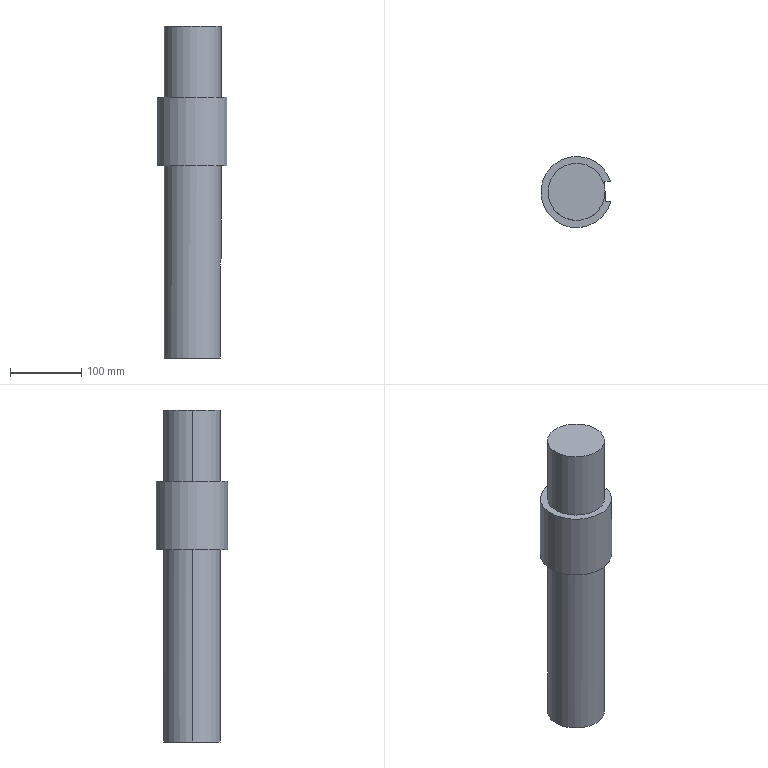Component | SolidWorks | 17WormGearShaft-1 | 1 solid | 16 faces | box 98.3 x 100 x 466 mm | volume 2562970 mm3 | plane 10 | cylinder 6 | commonest cylinder face diameters 80 x4 100 x1 22 x1
build123d program:
from build123d import *

# Parameters (mm, degrees)
SKETCH31_R          = 40
BOSS_EXTRUDE6_DEPTH = 466
BOSS_EXTRUDE9_START = -100
BOSS_EXTRUDE9_DEPTH = 96
CUT_EXTRUDE3_START  = 40
CUT_EXTRUDE3_DEPTH  = 9


with BuildPart() as part:
    # Sketch31 → Boss-Extrude6 (new body)
    with BuildSketch(Plane(origin=(0, 0, 0), x_dir=(0, 0, -1), z_dir=(1, 0, 0))):
        Circle(SKETCH31_R)
    extrude(amount=BOSS_EXTRUDE6_DEPTH)

    # Sketch32 → Boss-Extrude9 (add)
    with BuildSketch(Plane.ZY.offset(BOSS_EXTRUDE9_START)):
        with BuildLine():
            Line((48, 14), (40, 14))
            Line((40, 14), (40, -14))
            Line((40, -14), (48, -14))
            ThreePointArc((48, -14), (-50, 0), (48, 14))
        make_face()
    extrude(amount=-BOSS_EXTRUDE9_DEPTH)

    # Sketch33 → Cut-Extrude3 (cut)
    with BuildSketch(Plane.XY.offset(CUT_EXTRUDE3_START)):
        with BuildLine():
            Line((337, 11), (519.187, 11))
            ThreePointArc((519.187, 11), (530.187, 0), (519.187, -11))
            Line((519.187, -11), (337, -11))
            ThreePointArc((337, -11), (326, 0), (337, 11))
        make_face()
    extrude(amount=-CUT_EXTRUDE3_DEPTH, mode=Mode.SUBTRACT)


solid = part.part

# Placed as in the assembly
solid = solid.moved(Location((39.885, 141.809, 660), (-90, 88.714, 90)))
STEP:
#1=COLOUR_RGB('',0.7922,0.8196,0.9333);
#2=FILL_AREA_STYLE_COLOUR('',#1);
#3=FILL_AREA_STYLE('',(#2));
#4=SURFACE_STYLE_FILL_AREA(#3);
#5=SURFACE_SIDE_STYLE('',(#4));
#6=SURFACE_STYLE_USAGE(.BOTH.,#5);
#7=PRESENTATION_STYLE_ASSIGNMENT((#6));
#8=CARTESIAN_POINT('',(3.145,5.618,22.047));
#9=VERTEX_POINT('',#8);
#10=CARTESIAN_POINT('',(-0.004145,5.548,22.047));
#11=VERTEX_POINT('',#10);
#12=CARTESIAN_POINT('',(1.57,5.583,22.047));
#13=DIRECTION('',(0.,0.,1.));
#14=DIRECTION('',(0.9997,0.02244,0.));
#15=AXIS2_PLACEMENT_3D('',#12,#13,#14);
#16=CIRCLE('',#15,1.575);
#17=EDGE_CURVE('',#9,#11,#16,.T.);
#18=ORIENTED_EDGE('',*,*,#17,.T.);
#19=CARTESIAN_POINT('',(-0.004145,5.548,25.984));
#20=VERTEX_POINT('',#19);
#21=CARTESIAN_POINT('',(-0.004145,5.548,7.638));
#22=DIRECTION('',(0.,0.,1.));
#23=VECTOR('',#22,39.37);
#24=LINE('',#21,#23);
#25=EDGE_CURVE('',#11,#20,#24,.T.);
#26=ORIENTED_EDGE('',*,*,#25,.T.);
#27=CARTESIAN_POINT('',(3.145,5.618,25.984));
#28=VERTEX_POINT('',#27);
#29=CARTESIAN_POINT('',(1.57,5.583,25.984));
#30=DIRECTION('',(0.,0.,-1.));
#31=DIRECTION('',(-0.9997,-0.02244,0.));
#32=AXIS2_PLACEMENT_3D('',#29,#30,#31);
#33=CIRCLE('',#32,1.575);
#34=EDGE_CURVE('',#20,#28,#33,.T.);
#35=ORIENTED_EDGE('',*,*,#34,.T.);
#36=CARTESIAN_POINT('',(3.145,5.618,7.638));
#37=DIRECTION('',(0.,0.,1.));
#38=VECTOR('',#37,39.37);
#39=LINE('',#36,#38);
#40=EDGE_CURVE('',#9,#28,#39,.T.);
#41=ORIENTED_EDGE('',*,*,#40,.F.);
#42=EDGE_LOOP('',(#18,#26,#35,#41));
#43=FACE_OUTER_BOUND('',#42,.T.);
#44=CARTESIAN_POINT('',(1.57,5.583,7.638));
#45=DIRECTION('',(0.,0.,1.));
#46=DIRECTION('',(0.9997,0.02244,0.));
#47=AXIS2_PLACEMENT_3D('',#44,#45,#46);
#48=CYLINDRICAL_SURFACE('',#47,1.575);
#49=ADVANCED_FACE('',(#43),#48,.T.);
#50=CARTESIAN_POINT('',(-0.004145,5.548,7.638));
#51=VERTEX_POINT('',#50);
#52=CARTESIAN_POINT('',(3.074,6.05,7.638));
#53=VERTEX_POINT('',#52);
#54=CARTESIAN_POINT('',(1.57,5.583,7.638));
#55=DIRECTION('',(0.,0.,-1.));
#56=DIRECTION('',(-0.9997,-0.02244,0.));
#57=AXIS2_PLACEMENT_3D('',#54,#55,#56);
#58=CIRCLE('',#57,1.575);
#59=EDGE_CURVE('',#51,#53,#58,.T.);
#60=ORIENTED_EDGE('',*,*,#59,.F.);
#61=CARTESIAN_POINT('',(-0.004145,5.548,18.268));
#62=VERTEX_POINT('',#61);
#63=CARTESIAN_POINT('',(-0.004145,5.548,7.638));
#64=DIRECTION('',(0.,0.,1.));
#65=VECTOR('',#64,39.37);
#66=LINE('',#63,#65);
#67=EDGE_CURVE('',#51,#62,#66,.T.);
#68=ORIENTED_EDGE('',*,*,#67,.T.);
#69=CARTESIAN_POINT('',(3.145,5.618,18.268));
#70=VERTEX_POINT('',#69);
#71=CARTESIAN_POINT('',(1.57,5.583,18.268));
#72=DIRECTION('',(0.,0.,1.));
#73=DIRECTION('',(0.9997,0.02244,0.));
#74=AXIS2_PLACEMENT_3D('',#71,#72,#73);
#75=CIRCLE('',#74,1.575);
#76=EDGE_CURVE('',#70,#62,#75,.T.);
#77=ORIENTED_EDGE('',*,*,#76,.F.);
#78=CARTESIAN_POINT('',(3.145,5.618,13.15));
#79=VERTEX_POINT('',#78);
#80=CARTESIAN_POINT('',(3.145,5.618,7.638));
#81=DIRECTION('',(0.,0.,1.));
#82=VECTOR('',#81,39.37);
#83=LINE('',#80,#82);
#84=EDGE_CURVE('',#79,#70,#83,.T.);
#85=ORIENTED_EDGE('',*,*,#84,.F.);
#86=CARTESIAN_POINT('',(3.074,6.05,12.717));
#87=VERTEX_POINT('',#86);
#88=CARTESIAN_POINT('',(3.145,5.618,13.15));
#89=CARTESIAN_POINT('',(3.144,5.647,13.15));
#90=CARTESIAN_POINT('',(3.143,5.676,13.147));
#91=CARTESIAN_POINT('',(3.138,5.731,13.136));
#92=CARTESIAN_POINT('',(3.136,5.758,13.127));
#93=CARTESIAN_POINT('',(3.13,5.797,13.111));
#94=CARTESIAN_POINT('',(3.129,5.81,13.105));
#95=CARTESIAN_POINT('',(3.125,5.835,13.092));
#96=CARTESIAN_POINT('',(3.123,5.847,13.084));
#97=CARTESIAN_POINT('',(3.119,5.87,13.069));
#98=CARTESIAN_POINT('',(3.117,5.882,13.06));
#99=CARTESIAN_POINT('',(3.112,5.903,13.042));
#100=CARTESIAN_POINT('',(3.11,5.914,13.033));
#101=CARTESIAN_POINT('',(3.103,5.944,13.003));
#102=CARTESIAN_POINT('',(3.099,5.962,12.981));
#103=CARTESIAN_POINT('',(3.093,5.985,12.946));
#104=CARTESIAN_POINT('',(3.091,5.992,12.934));
#105=CARTESIAN_POINT('',(3.087,6.006,12.909));
#106=CARTESIAN_POINT('',(3.086,6.012,12.896));
#107=CARTESIAN_POINT('',(3.081,6.028,12.857));
#108=CARTESIAN_POINT('',(3.079,6.036,12.83));
#109=CARTESIAN_POINT('',(3.076,6.044,12.788));
#110=CARTESIAN_POINT('',(3.075,6.046,12.774));
#111=CARTESIAN_POINT('',(3.074,6.049,12.745));
#112=CARTESIAN_POINT('',(3.074,6.05,12.731));
#113=CARTESIAN_POINT('',(3.074,6.05,12.717));
#114=B_SPLINE_CURVE_WITH_KNOTS('',3,(#88,#89,#90,#91,#92,#93,#94,#95,#96,#97,#98,#99,#100,#101,#102,#103,#104,#105,#106,#107,#108,#109,#110,#111,#112,#113),.UNSPECIFIED.,.F.,.F.,(4,2,2,2,2,2,2,2,2,2,2,2,4),(0.01728,0.01944,0.0216,0.02268,0.02376,0.02484,0.02592,0.02807,0.02915,0.03023,0.03239,0.03347,0.03455),.UNSPECIFIED.);
#115=EDGE_CURVE('',#79,#87,#114,.T.);
#116=ORIENTED_EDGE('',*,*,#115,.T.);
#117=CARTESIAN_POINT('',(3.074,6.05,7.638));
#118=DIRECTION('',(0.,0.,-1.));
#119=VECTOR('',#118,39.37);
#120=LINE('',#117,#119);
#121=EDGE_CURVE('',#87,#53,#120,.T.);
#122=ORIENTED_EDGE('',*,*,#121,.T.);
#123=EDGE_LOOP('',(#60,#68,#77,#85,#116,#122));
#124=FACE_OUTER_BOUND('',#123,.T.);
#125=CARTESIAN_POINT('',(1.57,5.583,7.638));
#126=DIRECTION('',(0.,0.,1.));
#127=DIRECTION('',(0.9997,0.02244,0.));
#128=AXIS2_PLACEMENT_3D('',#125,#126,#127);
#129=CYLINDRICAL_SURFACE('',#128,1.575);
#130=ADVANCED_FACE('',(#124),#129,.T.);
#131=ORIENTED_EDGE('',*,*,#67,.F.);
#132=CARTESIAN_POINT('',(3.094,5.184,7.638));
#133=VERTEX_POINT('',#132);
#134=CARTESIAN_POINT('',(1.57,5.583,7.638));
#135=DIRECTION('',(0.,0.,-1.));
#136=DIRECTION('',(-0.9997,-0.02244,0.));
#137=AXIS2_PLACEMENT_3D('',#134,#135,#136);
#138=CIRCLE('',#137,1.575);
#139=EDGE_CURVE('',#133,#51,#138,.T.);
#140=ORIENTED_EDGE('',*,*,#139,.F.);
#141=CARTESIAN_POINT('',(3.094,5.184,12.717));
#142=VERTEX_POINT('',#141);
#143=CARTESIAN_POINT('',(3.094,5.184,7.638));
#144=DIRECTION('',(0.,0.,1.));
#145=VECTOR('',#144,39.37);
#146=LINE('',#143,#145);
#147=EDGE_CURVE('',#133,#142,#146,.T.);
#148=ORIENTED_EDGE('',*,*,#147,.T.);
#149=CARTESIAN_POINT('',(3.094,5.184,12.717));
#150=CARTESIAN_POINT('',(3.094,5.184,12.745));
#151=CARTESIAN_POINT('',(3.094,5.187,12.774));
#152=CARTESIAN_POINT('',(3.097,5.195,12.815));
#153=CARTESIAN_POINT('',(3.097,5.199,12.829));
#154=CARTESIAN_POINT('',(3.1,5.207,12.856));
#155=CARTESIAN_POINT('',(3.101,5.212,12.87));
#156=CARTESIAN_POINT('',(3.105,5.228,12.909));
#157=CARTESIAN_POINT('',(3.108,5.242,12.934));
#158=CARTESIAN_POINT('',(3.113,5.266,12.969));
#159=CARTESIAN_POINT('',(3.114,5.274,12.981));
#160=CARTESIAN_POINT('',(3.118,5.292,13.003));
#161=CARTESIAN_POINT('',(3.12,5.302,13.013));
#162=CARTESIAN_POINT('',(3.125,5.332,13.043));
#163=CARTESIAN_POINT('',(3.128,5.353,13.061));
#164=CARTESIAN_POINT('',(3.133,5.389,13.084));
#165=CARTESIAN_POINT('',(3.135,5.401,13.092));
#166=CARTESIAN_POINT('',(3.137,5.426,13.105));
#167=CARTESIAN_POINT('',(3.139,5.439,13.111));
#168=CARTESIAN_POINT('',(3.141,5.465,13.122));
#169=CARTESIAN_POINT('',(3.142,5.478,13.127));
#170=CARTESIAN_POINT('',(3.143,5.506,13.135));
#171=CARTESIAN_POINT('',(3.144,5.52,13.138));
#172=CARTESIAN_POINT('',(3.145,5.562,13.147));
#173=CARTESIAN_POINT('',(3.145,5.59,13.15));
#174=CARTESIAN_POINT('',(3.145,5.618,13.15));
#175=B_SPLINE_CURVE_WITH_KNOTS('',3,(#149,#150,#151,#152,#153,#154,#155,#156,#157,#158,#159,#160,#161,#162,#163,#164,#165,#166,#167,#168,#169,#170,#171,#172,#173,#174),.UNSPECIFIED.,.F.,.F.,(4,2,2,2,2,2,2,2,2,2,2,2,4),(0.,0.00216,0.003241,0.004321,0.006481,0.007562,0.008642,0.0108,0.01188,0.01296,0.01404,0.01512,0.01728),.UNSPECIFIED.);
#176=EDGE_CURVE('',#142,#79,#175,.T.);
#177=ORIENTED_EDGE('',*,*,#176,.T.);
#178=ORIENTED_EDGE('',*,*,#84,.T.);
#179=CARTESIAN_POINT('',(1.57,5.583,18.268));
#180=DIRECTION('',(0.,0.,1.));
#181=DIRECTION('',(0.9997,0.02244,0.));
#182=AXIS2_PLACEMENT_3D('',#179,#180,#181);
#183=CIRCLE('',#182,1.575);
#184=EDGE_CURVE('',#62,#70,#183,.T.);
#185=ORIENTED_EDGE('',*,*,#184,.F.);
#186=EDGE_LOOP('',(#131,#140,#148,#177,#178,#185));
#187=FACE_OUTER_BOUND('',#186,.T.);
#188=CARTESIAN_POINT('',(1.57,5.583,7.638));
#189=DIRECTION('',(0.,0.,1.));
#190=DIRECTION('',(0.9997,0.02244,0.));
#191=AXIS2_PLACEMENT_3D('',#188,#189,#190);
#192=CYLINDRICAL_SURFACE('',#191,1.575);
#193=ADVANCED_FACE('',(#187),#192,.T.);
#194=CARTESIAN_POINT('',(2.781,6.043,7.638));
#195=VERTEX_POINT('',#194);
#196=CARTESIAN_POINT('',(1.561,6.016,7.638));
#197=DIRECTION('',(0.9997,0.02244,0.));
#198=VECTOR('',#197,39.37);
#199=LINE('',#196,#198);
#200=EDGE_CURVE('',#195,#53,#199,.T.);
#201=ORIENTED_EDGE('',*,*,#200,.F.);
#202=CARTESIAN_POINT('',(2.8,5.177,7.638));
#203=VERTEX_POINT('',#202);
#204=CARTESIAN_POINT('',(2.79,5.61,7.638));
#205=DIRECTION('',(0.02244,-0.9997,0.));
#206=VECTOR('',#205,39.37);
#207=LINE('',#204,#206);
#208=EDGE_CURVE('',#195,#203,#207,.T.);
#209=ORIENTED_EDGE('',*,*,#208,.T.);
#210=CARTESIAN_POINT('',(1.58,5.15,7.638));
#211=DIRECTION('',(-0.9997,-0.02244,0.));
#212=VECTOR('',#211,39.37);
#213=LINE('',#210,#212);
#214=EDGE_CURVE('',#133,#203,#213,.T.);
#215=ORIENTED_EDGE('',*,*,#214,.F.);
#216=ORIENTED_EDGE('',*,*,#139,.T.);
#217=ORIENTED_EDGE('',*,*,#59,.T.);
#218=EDGE_LOOP('',(#201,#209,#215,#216,#217));
#219=FACE_OUTER_BOUND('',#218,.T.);
#220=CARTESIAN_POINT('',(1.57,5.583,7.638));
#221=DIRECTION('',(0.,0.,-1.));
#222=DIRECTION('',(-0.9997,-0.02244,0.));
#223=AXIS2_PLACEMENT_3D('',#220,#221,#222);
#224=PLANE('',#223);
#225=ADVANCED_FACE('',(#219),#224,.T.);
#226=CARTESIAN_POINT('',(3.157,5.067,18.268));
#227=VERTEX_POINT('',#226);
#228=CARTESIAN_POINT('',(3.132,6.169,18.268));
#229=DIRECTION('',(0.02244,-0.9997,0.));
#230=VECTOR('',#229,39.37);
#231=LINE('',#228,#230);
#232=EDGE_CURVE('',#70,#227,#231,.T.);
#233=ORIENTED_EDGE('',*,*,#232,.F.);
#234=CARTESIAN_POINT('',(3.132,6.169,18.268));
#235=VERTEX_POINT('',#234);
#236=CARTESIAN_POINT('',(3.132,6.169,18.268));
#237=DIRECTION('',(0.02244,-0.9997,0.));
#238=VECTOR('',#237,39.37);
#239=LINE('',#236,#238);
#240=EDGE_CURVE('',#235,#70,#239,.T.);
#241=ORIENTED_EDGE('',*,*,#240,.F.);
#242=CARTESIAN_POINT('',(3.132,6.169,22.047));
#243=VERTEX_POINT('',#242);
#244=CARTESIAN_POINT('',(3.132,6.169,18.268));
#245=DIRECTION('',(0.,0.,1.));
#246=VECTOR('',#245,39.37);
#247=LINE('',#244,#246);
#248=EDGE_CURVE('',#235,#243,#247,.T.);
#249=ORIENTED_EDGE('',*,*,#248,.T.);
#250=CARTESIAN_POINT('',(3.132,6.169,22.047));
#251=DIRECTION('',(0.02244,-0.9997,0.));
#252=VECTOR('',#251,39.37);
#253=LINE('',#250,#252);
#254=EDGE_CURVE('',#243,#9,#253,.T.);
#255=ORIENTED_EDGE('',*,*,#254,.T.);
#256=CARTESIAN_POINT('',(3.157,5.067,22.047));
#257=VERTEX_POINT('',#256);
#258=CARTESIAN_POINT('',(3.132,6.169,22.047));
#259=DIRECTION('',(0.02244,-0.9997,0.));
#260=VECTOR('',#259,39.37);
#261=LINE('',#258,#260);
#262=EDGE_CURVE('',#9,#257,#261,.T.);
#263=ORIENTED_EDGE('',*,*,#262,.T.);
#264=CARTESIAN_POINT('',(3.157,5.067,18.268));
#265=DIRECTION('',(0.,0.,1.));
#266=VECTOR('',#265,39.37);
#267=LINE('',#264,#266);
#268=EDGE_CURVE('',#227,#257,#267,.T.);
#269=ORIENTED_EDGE('',*,*,#268,.F.);
#270=EDGE_LOOP('',(#233,#241,#249,#255,#263,#269));
#271=FACE_OUTER_BOUND('',#270,.T.);
#272=CARTESIAN_POINT('',(3.132,6.169,18.268));
#273=DIRECTION('',(-0.9997,-0.02244,0.));
#274=DIRECTION('',(0.,0.,1.));
#275=AXIS2_PLACEMENT_3D('',#272,#273,#274);
#276=PLANE('',#275);
#277=ADVANCED_FACE('',(#271),#276,.F.);
#278=CARTESIAN_POINT('',(3.447,6.176,22.047));
#279=VERTEX_POINT('',#278);
#280=CARTESIAN_POINT('',(3.447,6.176,22.047));
#281=DIRECTION('',(-0.9997,-0.02244,0.));
#282=VECTOR('',#281,39.37);
#283=LINE('',#280,#282);
#284=EDGE_CURVE('',#279,#243,#283,.T.);
#285=ORIENTED_EDGE('',*,*,#284,.T.);
#286=ORIENTED_EDGE('',*,*,#248,.F.);
#287=CARTESIAN_POINT('',(3.447,6.176,18.268));
#288=VERTEX_POINT('',#287);
#289=CARTESIAN_POINT('',(3.447,6.176,18.268));
#290=DIRECTION('',(-0.9997,-0.02244,0.));
#291=VECTOR('',#290,39.37);
#292=LINE('',#289,#291);
#293=EDGE_CURVE('',#288,#235,#292,.T.);
#294=ORIENTED_EDGE('',*,*,#293,.F.);
#295=CARTESIAN_POINT('',(3.447,6.176,18.268));
#296=DIRECTION('',(0.,0.,1.));
#297=VECTOR('',#296,39.37);
#298=LINE('',#295,#297);
#299=EDGE_CURVE('',#288,#279,#298,.T.);
#300=ORIENTED_EDGE('',*,*,#299,.T.);
#301=EDGE_LOOP('',(#285,#286,#294,#300));
#302=FACE_OUTER_BOUND('',#301,.T.);
#303=CARTESIAN_POINT('',(3.447,6.176,18.268));
#304=DIRECTION('',(-0.02244,0.9997,0.));
#305=DIRECTION('',(0.9997,0.02244,0.));
#306=AXIS2_PLACEMENT_3D('',#303,#304,#305);
#307=PLANE('',#306);
#308=ADVANCED_FACE('',(#302),#307,.F.);
#309=CARTESIAN_POINT('',(3.472,5.074,22.047));
#310=VERTEX_POINT('',#309);
#311=CARTESIAN_POINT('',(3.472,5.074,22.047));
#312=DIRECTION('',(-0.9997,-0.02244,0.));
#313=VECTOR('',#312,39.37);
#314=LINE('',#311,#313);
#315=EDGE_CURVE('',#310,#257,#314,.T.);
#316=ORIENTED_EDGE('',*,*,#315,.F.);
#317=CARTESIAN_POINT('',(3.472,5.074,18.268));
#318=VERTEX_POINT('',#317);
#319=CARTESIAN_POINT('',(3.472,5.074,18.268));
#320=DIRECTION('',(0.,0.,1.));
#321=VECTOR('',#320,39.37);
#322=LINE('',#319,#321);
#323=EDGE_CURVE('',#318,#310,#322,.T.);
#324=ORIENTED_EDGE('',*,*,#323,.F.);
#325=CARTESIAN_POINT('',(3.472,5.074,18.268));
#326=DIRECTION('',(-0.9997,-0.02244,0.));
#327=VECTOR('',#326,39.37);
#328=LINE('',#325,#327);
#329=EDGE_CURVE('',#318,#227,#328,.T.);
#330=ORIENTED_EDGE('',*,*,#329,.T.);
#331=ORIENTED_EDGE('',*,*,#268,.T.);
#332=EDGE_LOOP('',(#316,#324,#330,#331));
#333=FACE_OUTER_BOUND('',#332,.T.);
#334=CARTESIAN_POINT('',(3.472,5.074,18.268));
#335=DIRECTION('',(-0.02244,0.9997,0.));
#336=DIRECTION('',(0.9997,0.02244,0.));
#337=AXIS2_PLACEMENT_3D('',#334,#335,#336);
#338=PLANE('',#337);
#339=ADVANCED_FACE('',(#333),#338,.T.);
#340=CARTESIAN_POINT('',(1.57,5.583,22.047));
#341=DIRECTION('',(0.,0.,1.));
#342=DIRECTION('',(0.9997,0.02244,0.));
#343=AXIS2_PLACEMENT_3D('',#340,#341,#342);
#344=CIRCLE('',#343,1.969);
#345=EDGE_CURVE('',#279,#310,#344,.T.);
#346=ORIENTED_EDGE('',*,*,#345,.F.);
#347=ORIENTED_EDGE('',*,*,#299,.F.);
#348=CARTESIAN_POINT('',(1.57,5.583,18.268));
#349=DIRECTION('',(0.,0.,1.));
#350=DIRECTION('',(0.9997,0.02244,0.));
#351=AXIS2_PLACEMENT_3D('',#348,#349,#350);
#352=CIRCLE('',#351,1.969);
#353=EDGE_CURVE('',#288,#318,#352,.T.);
#354=ORIENTED_EDGE('',*,*,#353,.T.);
#355=ORIENTED_EDGE('',*,*,#323,.T.);
#356=EDGE_LOOP('',(#346,#347,#354,#355));
#357=FACE_OUTER_BOUND('',#356,.T.);
#358=CARTESIAN_POINT('',(1.57,5.583,18.268));
#359=DIRECTION('',(0.,0.,1.));
#360=DIRECTION('',(0.9997,0.02244,0.));
#361=AXIS2_PLACEMENT_3D('',#358,#359,#360);
#362=CYLINDRICAL_SURFACE('',#361,1.969);
#363=ADVANCED_FACE('',(#357),#362,.T.);
#364=ORIENTED_EDGE('',*,*,#240,.T.);
#365=ORIENTED_EDGE('',*,*,#76,.T.);
#366=ORIENTED_EDGE('',*,*,#184,.T.);
#367=ORIENTED_EDGE('',*,*,#232,.T.);
#368=ORIENTED_EDGE('',*,*,#329,.F.);
#369=ORIENTED_EDGE('',*,*,#353,.F.);
#370=ORIENTED_EDGE('',*,*,#293,.T.);
#371=EDGE_LOOP('',(#364,#365,#366,#367,#368,#369,#370));
#372=FACE_OUTER_BOUND('',#371,.T.);
#373=CARTESIAN_POINT('',(1.57,5.583,18.268));
#374=DIRECTION('',(0.,0.,1.));
#375=DIRECTION('',(0.9997,0.02244,0.));
#376=AXIS2_PLACEMENT_3D('',#373,#374,#375);
#377=PLANE('',#376);
#378=ADVANCED_FACE('',(#372),#377,.F.);
#379=ORIENTED_EDGE('',*,*,#262,.F.);
#380=CARTESIAN_POINT('',(1.57,5.583,22.047));
#381=DIRECTION('',(0.,0.,1.));
#382=DIRECTION('',(0.9997,0.02244,0.));
#383=AXIS2_PLACEMENT_3D('',#380,#381,#382);
#384=CIRCLE('',#383,1.575);
#385=EDGE_CURVE('',#11,#9,#384,.T.);
#386=ORIENTED_EDGE('',*,*,#385,.F.);
#387=ORIENTED_EDGE('',*,*,#17,.F.);
#388=ORIENTED_EDGE('',*,*,#254,.F.);
#389=ORIENTED_EDGE('',*,*,#284,.F.);
#390=ORIENTED_EDGE('',*,*,#345,.T.);
#391=ORIENTED_EDGE('',*,*,#315,.T.);
#392=EDGE_LOOP('',(#379,#386,#387,#388,#389,#390,#391));
#393=FACE_OUTER_BOUND('',#392,.T.);
#394=CARTESIAN_POINT('',(1.57,5.583,22.047));
#395=DIRECTION('',(0.,0.,1.));
#396=DIRECTION('',(0.9997,0.02244,0.));
#397=AXIS2_PLACEMENT_3D('',#394,#395,#396);
#398=PLANE('',#397);
#399=ADVANCED_FACE('',(#393),#398,.T.);
#400=CARTESIAN_POINT('',(1.57,5.583,25.984));
#401=DIRECTION('',(0.,0.,-1.));
#402=DIRECTION('',(-0.9997,-0.02244,0.));
#403=AXIS2_PLACEMENT_3D('',#400,#401,#402);
#404=CIRCLE('',#403,1.575);
#405=EDGE_CURVE('',#28,#20,#404,.T.);
#406=ORIENTED_EDGE('',*,*,#405,.F.);
#407=ORIENTED_EDGE('',*,*,#34,.F.);
#408=EDGE_LOOP('',(#406,#407));
#409=FACE_OUTER_BOUND('',#408,.T.);
#410=CARTESIAN_POINT('',(1.57,5.583,25.984));
#411=DIRECTION('',(0.,0.,-1.));
#412=DIRECTION('',(-0.9997,-0.02244,0.));
#413=AXIS2_PLACEMENT_3D('',#410,#411,#412);
#414=PLANE('',#413);
#415=ADVANCED_FACE('',(#409),#414,.F.);
#416=ORIENTED_EDGE('',*,*,#25,.F.);
#417=ORIENTED_EDGE('',*,*,#385,.T.);
#418=ORIENTED_EDGE('',*,*,#40,.T.);
#419=ORIENTED_EDGE('',*,*,#405,.T.);
#420=EDGE_LOOP('',(#416,#417,#418,#419));
#421=FACE_OUTER_BOUND('',#420,.T.);
#422=CARTESIAN_POINT('',(1.57,5.583,7.638));
#423=DIRECTION('',(0.,0.,1.));
#424=DIRECTION('',(0.9997,0.02244,0.));
#425=AXIS2_PLACEMENT_3D('',#422,#423,#424);
#426=CYLINDRICAL_SURFACE('',#425,1.575);
#427=ADVANCED_FACE('',(#421),#426,.T.);
#428=CARTESIAN_POINT('',(2.8,5.177,12.717));
#429=VERTEX_POINT('',#428);
#430=CARTESIAN_POINT('',(2.8,5.177,12.717));
#431=DIRECTION('',(0.9997,0.02244,0.));
#432=VECTOR('',#431,39.37);
#433=LINE('',#430,#432);
#434=EDGE_CURVE('',#429,#142,#433,.T.);
#435=ORIENTED_EDGE('',*,*,#434,.F.);
#436=CARTESIAN_POINT('',(2.781,6.043,12.717));
#437=VERTEX_POINT('',#436);
#438=CARTESIAN_POINT('',(2.79,5.61,12.717));
#439=DIRECTION('',(0.9997,0.02244,0.));
#440=DIRECTION('',(0.,0.,-1.));
#441=AXIS2_PLACEMENT_3D('',#438,#439,#440);
#442=CIRCLE('',#441,0.4331);
#443=EDGE_CURVE('',#437,#429,#442,.T.);
#444=ORIENTED_EDGE('',*,*,#443,.F.);
#445=CARTESIAN_POINT('',(2.781,6.043,12.717));
#446=DIRECTION('',(0.9997,0.02244,0.));
#447=VECTOR('',#446,39.37);
#448=LINE('',#445,#447);
#449=EDGE_CURVE('',#437,#87,#448,.T.);
#450=ORIENTED_EDGE('',*,*,#449,.T.);
#451=ORIENTED_EDGE('',*,*,#115,.F.);
#452=ORIENTED_EDGE('',*,*,#176,.F.);
#453=EDGE_LOOP('',(#435,#444,#450,#451,#452));
#454=FACE_OUTER_BOUND('',#453,.T.);
#455=CARTESIAN_POINT('',(2.79,5.61,12.717));
#456=DIRECTION('',(0.9997,0.02244,0.));
#457=DIRECTION('',(0.,0.,-1.));
#458=AXIS2_PLACEMENT_3D('',#455,#456,#457);
#459=CYLINDRICAL_SURFACE('',#458,0.4331);
#460=ADVANCED_FACE('',(#454),#459,.F.);
#461=ORIENTED_EDGE('',*,*,#449,.F.);
#462=CARTESIAN_POINT('',(2.781,6.043,12.717));
#463=DIRECTION('',(0.,0.,1.));
#464=VECTOR('',#463,39.37);
#465=LINE('',#462,#464);
#466=EDGE_CURVE('',#195,#437,#465,.T.);
#467=ORIENTED_EDGE('',*,*,#466,.F.);
#468=ORIENTED_EDGE('',*,*,#200,.T.);
#469=ORIENTED_EDGE('',*,*,#121,.F.);
#470=EDGE_LOOP('',(#461,#467,#468,#469));
#471=FACE_OUTER_BOUND('',#470,.T.);
#472=CARTESIAN_POINT('',(2.781,6.043,12.717));
#473=DIRECTION('',(-0.02244,0.9997,0.));
#474=DIRECTION('',(0.9997,0.02244,0.));
#475=AXIS2_PLACEMENT_3D('',#472,#473,#474);
#476=PLANE('',#475);
#477=ADVANCED_FACE('',(#471),#476,.F.);
#478=ORIENTED_EDGE('',*,*,#214,.T.);
#479=CARTESIAN_POINT('',(2.8,5.177,12.717));
#480=DIRECTION('',(0.,0.,-1.));
#481=VECTOR('',#480,39.37);
#482=LINE('',#479,#481);
#483=EDGE_CURVE('',#429,#203,#482,.T.);
#484=ORIENTED_EDGE('',*,*,#483,.F.);
#485=ORIENTED_EDGE('',*,*,#434,.T.);
#486=ORIENTED_EDGE('',*,*,#147,.F.);
#487=EDGE_LOOP('',(#478,#484,#485,#486));
#488=FACE_OUTER_BOUND('',#487,.T.);
#489=CARTESIAN_POINT('',(2.8,5.177,12.717));
#490=DIRECTION('',(0.02244,-0.9997,0.));
#491=DIRECTION('',(-0.9997,-0.02244,0.));
#492=AXIS2_PLACEMENT_3D('',#489,#490,#491);
#493=PLANE('',#492);
#494=ADVANCED_FACE('',(#488),#493,.F.);
#495=ORIENTED_EDGE('',*,*,#466,.T.);
#496=ORIENTED_EDGE('',*,*,#443,.T.);
#497=ORIENTED_EDGE('',*,*,#483,.T.);
#498=ORIENTED_EDGE('',*,*,#208,.F.);
#499=EDGE_LOOP('',(#495,#496,#497,#498));
#500=FACE_OUTER_BOUND('',#499,.T.);
#501=CARTESIAN_POINT('',(2.79,5.61,12.717));
#502=DIRECTION('',(0.9997,0.02244,0.));
#503=DIRECTION('',(0.,0.,-1.));
#504=AXIS2_PLACEMENT_3D('',#501,#502,#503);
#505=PLANE('',#504);
#506=ADVANCED_FACE('',(#500),#505,.T.);
#507=CLOSED_SHELL('',(#49,#130,#193,#225,#277,#308,#339,#363,#378,#399,#415,#427,#460,#477,#494,#506));
#508=MANIFOLD_SOLID_BREP('',#507);
#509=STYLED_ITEM('',(#7),#508);
#510=PRESENTATION_LAYER_ASSIGNMENT('','',(#509));
#511=(LENGTH_UNIT()NAMED_UNIT(*)SI_UNIT($,.METRE.));
#512=LENGTH_MEASURE_WITH_UNIT(LENGTH_MEASURE(0.0254),#511);
#513=DIMENSIONAL_EXPONENTS(1.,0.,0.,0.,0.,0.,0.);
#514=(CONVERSION_BASED_UNIT('',#512)LENGTH_UNIT()NAMED_UNIT(#513));
#515=UNCERTAINTY_MEASURE_WITH_UNIT(LENGTH_MEASURE(0.00001),#514,'','');
#516=(NAMED_UNIT(*)PLANE_ANGLE_UNIT()SI_UNIT($,.RADIAN.));
#517=(NAMED_UNIT(*)SI_UNIT($,.STERADIAN.)SOLID_ANGLE_UNIT());
#518=(GEOMETRIC_REPRESENTATION_CONTEXT(3)GLOBAL_UNCERTAINTY_ASSIGNED_CONTEXT((#515))GLOBAL_UNIT_ASSIGNED_CONTEXT((#514,#516,#517))REPRESENTATION_CONTEXT('',''));
#519=MECHANICAL_DESIGN_GEOMETRIC_PRESENTATION_REPRESENTATION('',(#509),#518);
#520=CARTESIAN_POINT('',(0.,0.,0.));
#521=DIRECTION('',(0.,0.,1.));
#522=DIRECTION('',(1.,0.,0.));
#523=AXIS2_PLACEMENT_3D('',#520,#521,#522);
#524=(LENGTH_UNIT()NAMED_UNIT(*)SI_UNIT($,.METRE.));
#525=LENGTH_MEASURE_WITH_UNIT(LENGTH_MEASURE(0.0254),#524);
#526=DIMENSIONAL_EXPONENTS(1.,0.,0.,0.,0.,0.,0.);
#527=(CONVERSION_BASED_UNIT('',#525)LENGTH_UNIT()NAMED_UNIT(#526));
#528=UNCERTAINTY_MEASURE_WITH_UNIT(LENGTH_MEASURE(0.00001),#527,'','');
#529=(NAMED_UNIT(*)PLANE_ANGLE_UNIT()SI_UNIT($,.RADIAN.));
#530=(NAMED_UNIT(*)SI_UNIT($,.STERADIAN.)SOLID_ANGLE_UNIT());
#531=(GEOMETRIC_REPRESENTATION_CONTEXT(3)GLOBAL_UNCERTAINTY_ASSIGNED_CONTEXT((#528))GLOBAL_UNIT_ASSIGNED_CONTEXT((#527,#529,#530))REPRESENTATION_CONTEXT('',''));
#532=ADVANCED_BREP_SHAPE_REPRESENTATION('',(#508,#523),#531);